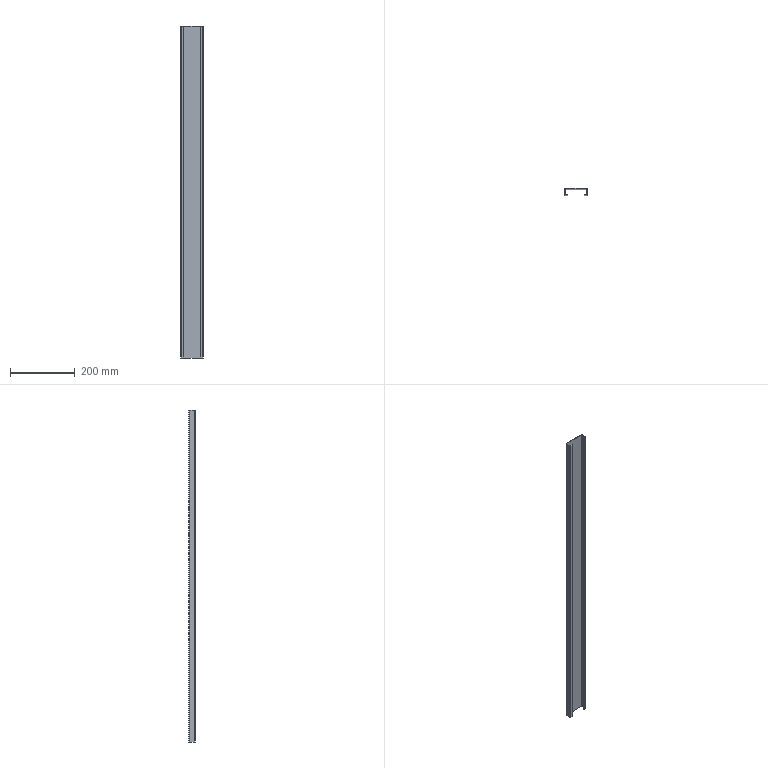Component | SolidWorks | MiddleColumn3-1 | 1 solid | 38 faces | box 70 x 20 x 1025 mm | volume 184711 mm3 | plane 30 | cylinder 8 | commonest cylinder face diameters 3 x4 6 x4
STEP:
#1=COLOUR_RGB('',0.7922,0.8196,0.9333);
#2=FILL_AREA_STYLE_COLOUR('',#1);
#3=FILL_AREA_STYLE('',(#2));
#4=SURFACE_STYLE_FILL_AREA(#3);
#5=SURFACE_SIDE_STYLE('',(#4));
#6=SURFACE_STYLE_USAGE(.BOTH.,#5);
#7=PRESENTATION_STYLE_ASSIGNMENT((#6));
#8=CARTESIAN_POINT('',(-11.614,-13.549,0.9843));
#9=VERTEX_POINT('',#8);
#10=CARTESIAN_POINT('',(-11.614,-13.49,0.9843));
#11=VERTEX_POINT('',#10);
#12=CARTESIAN_POINT('',(-11.614,-13.549,0.9843));
#13=DIRECTION('',(-0.,1.,0.));
#14=VECTOR('',#13,39.37);
#15=LINE('',#12,#14);
#16=EDGE_CURVE('',#9,#11,#15,.T.);
#17=ORIENTED_EDGE('',*,*,#16,.F.);
#18=CARTESIAN_POINT('',(-11.732,-13.431,0.9843));
#19=VERTEX_POINT('',#18);
#20=CARTESIAN_POINT('',(-11.614,-13.431,0.9843));
#21=DIRECTION('',(0.,0.,-1.));
#22=DIRECTION('',(0.,-1.,-0.));
#23=AXIS2_PLACEMENT_3D('',#20,#21,#22);
#24=CIRCLE('',#23,0.1181);
#25=EDGE_CURVE('',#9,#19,#24,.T.);
#26=ORIENTED_EDGE('',*,*,#25,.T.);
#27=CARTESIAN_POINT('',(-11.673,-13.431,0.9843));
#28=VERTEX_POINT('',#27);
#29=CARTESIAN_POINT('',(-11.673,-13.431,0.9843));
#30=DIRECTION('',(-1.,-0.,-0.));
#31=VECTOR('',#30,39.37);
#32=LINE('',#29,#31);
#33=EDGE_CURVE('',#28,#19,#32,.T.);
#34=ORIENTED_EDGE('',*,*,#33,.F.);
#35=CARTESIAN_POINT('',(-11.614,-13.431,0.9843));
#36=DIRECTION('',(0.,0.,-1.));
#37=DIRECTION('',(1.,0.,0.));
#38=AXIS2_PLACEMENT_3D('',#35,#36,#37);
#39=CIRCLE('',#38,0.05906);
#40=EDGE_CURVE('',#11,#28,#39,.T.);
#41=ORIENTED_EDGE('',*,*,#40,.F.);
#42=EDGE_LOOP('',(#17,#26,#34,#41));
#43=FACE_OUTER_BOUND('',#42,.T.);
#44=CARTESIAN_POINT('',(-11.614,-13.549,0.9843));
#45=DIRECTION('',(0.,0.,-1.));
#46=DIRECTION('',(-0.,1.,0.));
#47=AXIS2_PLACEMENT_3D('',#44,#45,#46);
#48=PLANE('',#47);
#49=ADVANCED_FACE('',(#43),#48,.T.);
#50=CARTESIAN_POINT('',(-11.339,-13.549,0.9843));
#51=VERTEX_POINT('',#50);
#52=CARTESIAN_POINT('',(-11.339,-13.549,0.9843));
#53=DIRECTION('',(-1.,-0.,-0.));
#54=VECTOR('',#53,39.37);
#55=LINE('',#52,#54);
#56=EDGE_CURVE('',#51,#9,#55,.T.);
#57=ORIENTED_EDGE('',*,*,#56,.T.);
#58=ORIENTED_EDGE('',*,*,#16,.T.);
#59=CARTESIAN_POINT('',(-11.339,-13.49,0.9843));
#60=VERTEX_POINT('',#59);
#61=CARTESIAN_POINT('',(-11.339,-13.49,0.9843));
#62=DIRECTION('',(-1.,-0.,-0.));
#63=VECTOR('',#62,39.37);
#64=LINE('',#61,#63);
#65=EDGE_CURVE('',#60,#11,#64,.T.);
#66=ORIENTED_EDGE('',*,*,#65,.F.);
#67=CARTESIAN_POINT('',(-11.339,-13.549,0.9843));
#68=DIRECTION('',(-0.,1.,0.));
#69=VECTOR('',#68,39.37);
#70=LINE('',#67,#69);
#71=EDGE_CURVE('',#51,#60,#70,.T.);
#72=ORIENTED_EDGE('',*,*,#71,.F.);
#73=EDGE_LOOP('',(#57,#58,#66,#72));
#74=FACE_OUTER_BOUND('',#73,.T.);
#75=CARTESIAN_POINT('',(-11.673,-13.431,0.9843));
#76=DIRECTION('',(0.,0.,-1.));
#77=DIRECTION('',(-0.,1.,0.));
#78=AXIS2_PLACEMENT_3D('',#75,#76,#77);
#79=PLANE('',#78);
#80=ADVANCED_FACE('',(#74),#79,.T.);
#81=CARTESIAN_POINT('',(-11.732,-13.431,41.339));
#82=VERTEX_POINT('',#81);
#83=CARTESIAN_POINT('',(-11.673,-13.431,41.339));
#84=VERTEX_POINT('',#83);
#85=CARTESIAN_POINT('',(-11.732,-13.431,41.339));
#86=DIRECTION('',(1.,0.,0.));
#87=VECTOR('',#86,39.37);
#88=LINE('',#85,#87);
#89=EDGE_CURVE('',#82,#84,#88,.T.);
#90=ORIENTED_EDGE('',*,*,#89,.F.);
#91=CARTESIAN_POINT('',(-11.614,-13.549,41.339));
#92=VERTEX_POINT('',#91);
#93=CARTESIAN_POINT('',(-11.614,-13.431,41.339));
#94=DIRECTION('',(0.,0.,-1.));
#95=DIRECTION('',(0.,-1.,0.));
#96=AXIS2_PLACEMENT_3D('',#93,#94,#95);
#97=CIRCLE('',#96,0.1181);
#98=EDGE_CURVE('',#92,#82,#97,.T.);
#99=ORIENTED_EDGE('',*,*,#98,.F.);
#100=CARTESIAN_POINT('',(-11.614,-13.49,41.339));
#101=VERTEX_POINT('',#100);
#102=CARTESIAN_POINT('',(-11.614,-13.49,41.339));
#103=DIRECTION('',(0.,-1.,-0.));
#104=VECTOR('',#103,39.37);
#105=LINE('',#102,#104);
#106=EDGE_CURVE('',#101,#92,#105,.T.);
#107=ORIENTED_EDGE('',*,*,#106,.F.);
#108=CARTESIAN_POINT('',(-11.614,-13.431,41.339));
#109=DIRECTION('',(0.,0.,-1.));
#110=DIRECTION('',(1.,0.,0.));
#111=AXIS2_PLACEMENT_3D('',#108,#109,#110);
#112=CIRCLE('',#111,0.05906);
#113=EDGE_CURVE('',#101,#84,#112,.T.);
#114=ORIENTED_EDGE('',*,*,#113,.T.);
#115=EDGE_LOOP('',(#90,#99,#107,#114));
#116=FACE_OUTER_BOUND('',#115,.T.);
#117=CARTESIAN_POINT('',(-11.732,-13.431,41.339));
#118=DIRECTION('',(-0.,-0.,1.));
#119=DIRECTION('',(0.,-1.,-0.));
#120=AXIS2_PLACEMENT_3D('',#117,#118,#119);
#121=PLANE('',#120);
#122=ADVANCED_FACE('',(#116),#121,.T.);
#123=CARTESIAN_POINT('',(-11.732,-12.88,41.339));
#124=VERTEX_POINT('',#123);
#125=CARTESIAN_POINT('',(-11.732,-13.549,41.339));
#126=DIRECTION('',(-0.,1.,0.));
#127=VECTOR('',#126,39.37);
#128=LINE('',#125,#127);
#129=EDGE_CURVE('',#82,#124,#128,.T.);
#130=ORIENTED_EDGE('',*,*,#129,.F.);
#131=ORIENTED_EDGE('',*,*,#89,.T.);
#132=CARTESIAN_POINT('',(-11.673,-12.88,41.339));
#133=VERTEX_POINT('',#132);
#134=CARTESIAN_POINT('',(-11.673,-13.549,41.339));
#135=DIRECTION('',(-0.,1.,0.));
#136=VECTOR('',#135,39.37);
#137=LINE('',#134,#136);
#138=EDGE_CURVE('',#84,#133,#137,.T.);
#139=ORIENTED_EDGE('',*,*,#138,.T.);
#140=CARTESIAN_POINT('',(-11.673,-12.88,41.339));
#141=DIRECTION('',(-1.,0.,-0.));
#142=VECTOR('',#141,39.37);
#143=LINE('',#140,#142);
#144=EDGE_CURVE('',#133,#124,#143,.T.);
#145=ORIENTED_EDGE('',*,*,#144,.T.);
#146=EDGE_LOOP('',(#130,#131,#139,#145));
#147=FACE_OUTER_BOUND('',#146,.T.);
#148=CARTESIAN_POINT('',(-11.614,-13.49,41.339));
#149=DIRECTION('',(-0.,-0.,1.));
#150=DIRECTION('',(0.,-1.,-0.));
#151=AXIS2_PLACEMENT_3D('',#148,#149,#150);
#152=PLANE('',#151);
#153=ADVANCED_FACE('',(#147),#152,.T.);
#154=CARTESIAN_POINT('',(-11.732,-12.88,0.9843));
#155=VERTEX_POINT('',#154);
#156=CARTESIAN_POINT('',(-11.673,-12.88,0.9843));
#157=VERTEX_POINT('',#156);
#158=CARTESIAN_POINT('',(-11.732,-12.88,0.9843));
#159=DIRECTION('',(1.,-0.,0.));
#160=VECTOR('',#159,39.37);
#161=LINE('',#158,#160);
#162=EDGE_CURVE('',#155,#157,#161,.T.);
#163=ORIENTED_EDGE('',*,*,#162,.F.);
#164=CARTESIAN_POINT('',(-11.614,-12.762,0.9843));
#165=VERTEX_POINT('',#164);
#166=CARTESIAN_POINT('',(-11.614,-12.88,0.9843));
#167=DIRECTION('',(0.,0.,-1.));
#168=DIRECTION('',(0.,-1.,-0.));
#169=AXIS2_PLACEMENT_3D('',#166,#167,#168);
#170=CIRCLE('',#169,0.1181);
#171=EDGE_CURVE('',#155,#165,#170,.T.);
#172=ORIENTED_EDGE('',*,*,#171,.T.);
#173=CARTESIAN_POINT('',(-11.614,-12.821,0.9843));
#174=VERTEX_POINT('',#173);
#175=CARTESIAN_POINT('',(-11.614,-12.821,0.9843));
#176=DIRECTION('',(-0.,1.,0.));
#177=VECTOR('',#176,39.37);
#178=LINE('',#175,#177);
#179=EDGE_CURVE('',#174,#165,#178,.T.);
#180=ORIENTED_EDGE('',*,*,#179,.F.);
#181=CARTESIAN_POINT('',(-11.614,-12.88,0.9843));
#182=DIRECTION('',(0.,0.,-1.));
#183=DIRECTION('',(1.,0.,0.));
#184=AXIS2_PLACEMENT_3D('',#181,#182,#183);
#185=CIRCLE('',#184,0.05906);
#186=EDGE_CURVE('',#157,#174,#185,.T.);
#187=ORIENTED_EDGE('',*,*,#186,.F.);
#188=EDGE_LOOP('',(#163,#172,#180,#187));
#189=FACE_OUTER_BOUND('',#188,.T.);
#190=CARTESIAN_POINT('',(-11.732,-12.88,0.9843));
#191=DIRECTION('',(0.,0.,-1.));
#192=DIRECTION('',(-0.,1.,0.));
#193=AXIS2_PLACEMENT_3D('',#190,#191,#192);
#194=PLANE('',#193);
#195=ADVANCED_FACE('',(#189),#194,.T.);
#196=CARTESIAN_POINT('',(-11.732,-13.549,0.9843));
#197=DIRECTION('',(-0.,1.,0.));
#198=VECTOR('',#197,39.37);
#199=LINE('',#196,#198);
#200=EDGE_CURVE('',#19,#155,#199,.T.);
#201=ORIENTED_EDGE('',*,*,#200,.T.);
#202=ORIENTED_EDGE('',*,*,#162,.T.);
#203=CARTESIAN_POINT('',(-11.673,-13.549,0.9843));
#204=DIRECTION('',(-0.,1.,0.));
#205=VECTOR('',#204,39.37);
#206=LINE('',#203,#205);
#207=EDGE_CURVE('',#28,#157,#206,.T.);
#208=ORIENTED_EDGE('',*,*,#207,.F.);
#209=ORIENTED_EDGE('',*,*,#33,.T.);
#210=EDGE_LOOP('',(#201,#202,#208,#209));
#211=FACE_OUTER_BOUND('',#210,.T.);
#212=CARTESIAN_POINT('',(-11.614,-12.821,0.9843));
#213=DIRECTION('',(0.,0.,-1.));
#214=DIRECTION('',(-0.,1.,0.));
#215=AXIS2_PLACEMENT_3D('',#212,#213,#214);
#216=PLANE('',#215);
#217=ADVANCED_FACE('',(#211),#216,.T.);
#218=CARTESIAN_POINT('',(-11.614,-12.762,41.339));
#219=VERTEX_POINT('',#218);
#220=CARTESIAN_POINT('',(-11.614,-12.821,41.339));
#221=VERTEX_POINT('',#220);
#222=CARTESIAN_POINT('',(-11.614,-12.762,41.339));
#223=DIRECTION('',(0.,-1.,-0.));
#224=VECTOR('',#223,39.37);
#225=LINE('',#222,#224);
#226=EDGE_CURVE('',#219,#221,#225,.T.);
#227=ORIENTED_EDGE('',*,*,#226,.F.);
#228=CARTESIAN_POINT('',(-11.614,-12.88,41.339));
#229=DIRECTION('',(0.,0.,-1.));
#230=DIRECTION('',(0.,-1.,0.));
#231=AXIS2_PLACEMENT_3D('',#228,#229,#230);
#232=CIRCLE('',#231,0.1181);
#233=EDGE_CURVE('',#124,#219,#232,.T.);
#234=ORIENTED_EDGE('',*,*,#233,.F.);
#235=ORIENTED_EDGE('',*,*,#144,.F.);
#236=CARTESIAN_POINT('',(-11.614,-12.88,41.339));
#237=DIRECTION('',(0.,0.,-1.));
#238=DIRECTION('',(1.,0.,0.));
#239=AXIS2_PLACEMENT_3D('',#236,#237,#238);
#240=CIRCLE('',#239,0.05906);
#241=EDGE_CURVE('',#133,#221,#240,.T.);
#242=ORIENTED_EDGE('',*,*,#241,.T.);
#243=EDGE_LOOP('',(#227,#234,#235,#242));
#244=FACE_OUTER_BOUND('',#243,.T.);
#245=CARTESIAN_POINT('',(-11.614,-12.762,41.339));
#246=DIRECTION('',(-0.,-0.,1.));
#247=DIRECTION('',(0.,-1.,-0.));
#248=AXIS2_PLACEMENT_3D('',#245,#246,#247);
#249=PLANE('',#248);
#250=ADVANCED_FACE('',(#244),#249,.T.);
#251=CARTESIAN_POINT('',(-9.095,-12.762,41.339));
#252=VERTEX_POINT('',#251);
#253=CARTESIAN_POINT('',(-11.732,-12.762,41.339));
#254=DIRECTION('',(1.,-0.,0.));
#255=VECTOR('',#254,39.37);
#256=LINE('',#253,#255);
#257=EDGE_CURVE('',#219,#252,#256,.T.);
#258=ORIENTED_EDGE('',*,*,#257,.F.);
#259=ORIENTED_EDGE('',*,*,#226,.T.);
#260=CARTESIAN_POINT('',(-9.095,-12.821,41.339));
#261=VERTEX_POINT('',#260);
#262=CARTESIAN_POINT('',(-11.732,-12.821,41.339));
#263=DIRECTION('',(1.,-0.,0.));
#264=VECTOR('',#263,39.37);
#265=LINE('',#262,#264);
#266=EDGE_CURVE('',#221,#261,#265,.T.);
#267=ORIENTED_EDGE('',*,*,#266,.T.);
#268=CARTESIAN_POINT('',(-9.095,-12.821,41.339));
#269=DIRECTION('',(-0.,1.,0.));
#270=VECTOR('',#269,39.37);
#271=LINE('',#268,#270);
#272=EDGE_CURVE('',#261,#252,#271,.T.);
#273=ORIENTED_EDGE('',*,*,#272,.T.);
#274=EDGE_LOOP('',(#258,#259,#267,#273));
#275=FACE_OUTER_BOUND('',#274,.T.);
#276=CARTESIAN_POINT('',(-11.673,-12.88,41.339));
#277=DIRECTION('',(-0.,-0.,1.));
#278=DIRECTION('',(0.,-1.,-0.));
#279=AXIS2_PLACEMENT_3D('',#276,#277,#278);
#280=PLANE('',#279);
#281=ADVANCED_FACE('',(#275),#280,.T.);
#282=CARTESIAN_POINT('',(-9.095,-12.762,0.9843));
#283=VERTEX_POINT('',#282);
#284=CARTESIAN_POINT('',(-9.095,-12.821,0.9843));
#285=VERTEX_POINT('',#284);
#286=CARTESIAN_POINT('',(-9.095,-12.762,0.9843));
#287=DIRECTION('',(0.,-1.,-0.));
#288=VECTOR('',#287,39.37);
#289=LINE('',#286,#288);
#290=EDGE_CURVE('',#283,#285,#289,.T.);
#291=ORIENTED_EDGE('',*,*,#290,.F.);
#292=CARTESIAN_POINT('',(-8.976,-12.88,0.9843));
#293=VERTEX_POINT('',#292);
#294=CARTESIAN_POINT('',(-9.095,-12.88,0.9843));
#295=DIRECTION('',(0.,0.,-1.));
#296=DIRECTION('',(0.,-1.,-0.));
#297=AXIS2_PLACEMENT_3D('',#294,#295,#296);
#298=CIRCLE('',#297,0.1181);
#299=EDGE_CURVE('',#283,#293,#298,.T.);
#300=ORIENTED_EDGE('',*,*,#299,.T.);
#301=CARTESIAN_POINT('',(-9.036,-12.88,0.9843));
#302=VERTEX_POINT('',#301);
#303=CARTESIAN_POINT('',(-9.036,-12.88,0.9843));
#304=DIRECTION('',(1.,0.,0.));
#305=VECTOR('',#304,39.37);
#306=LINE('',#303,#305);
#307=EDGE_CURVE('',#302,#293,#306,.T.);
#308=ORIENTED_EDGE('',*,*,#307,.F.);
#309=CARTESIAN_POINT('',(-9.095,-12.88,0.9843));
#310=DIRECTION('',(0.,0.,-1.));
#311=DIRECTION('',(1.,0.,0.));
#312=AXIS2_PLACEMENT_3D('',#309,#310,#311);
#313=CIRCLE('',#312,0.05906);
#314=EDGE_CURVE('',#285,#302,#313,.T.);
#315=ORIENTED_EDGE('',*,*,#314,.F.);
#316=EDGE_LOOP('',(#291,#300,#308,#315));
#317=FACE_OUTER_BOUND('',#316,.T.);
#318=CARTESIAN_POINT('',(-9.095,-12.762,0.9843));
#319=DIRECTION('',(0.,0.,-1.));
#320=DIRECTION('',(-0.,1.,0.));
#321=AXIS2_PLACEMENT_3D('',#318,#319,#320);
#322=PLANE('',#321);
#323=ADVANCED_FACE('',(#317),#322,.T.);
#324=CARTESIAN_POINT('',(-11.732,-12.762,0.9843));
#325=DIRECTION('',(1.,-0.,0.));
#326=VECTOR('',#325,39.37);
#327=LINE('',#324,#326);
#328=EDGE_CURVE('',#165,#283,#327,.T.);
#329=ORIENTED_EDGE('',*,*,#328,.T.);
#330=ORIENTED_EDGE('',*,*,#290,.T.);
#331=CARTESIAN_POINT('',(-11.732,-12.821,0.9843));
#332=DIRECTION('',(1.,-0.,0.));
#333=VECTOR('',#332,39.37);
#334=LINE('',#331,#333);
#335=EDGE_CURVE('',#174,#285,#334,.T.);
#336=ORIENTED_EDGE('',*,*,#335,.F.);
#337=ORIENTED_EDGE('',*,*,#179,.T.);
#338=EDGE_LOOP('',(#329,#330,#336,#337));
#339=FACE_OUTER_BOUND('',#338,.T.);
#340=CARTESIAN_POINT('',(-9.036,-12.88,0.9843));
#341=DIRECTION('',(0.,0.,-1.));
#342=DIRECTION('',(-0.,1.,0.));
#343=AXIS2_PLACEMENT_3D('',#340,#341,#342);
#344=PLANE('',#343);
#345=ADVANCED_FACE('',(#339),#344,.T.);
#346=CARTESIAN_POINT('',(-8.976,-12.88,41.339));
#347=VERTEX_POINT('',#346);
#348=CARTESIAN_POINT('',(-9.036,-12.88,41.339));
#349=VERTEX_POINT('',#348);
#350=CARTESIAN_POINT('',(-8.976,-12.88,41.339));
#351=DIRECTION('',(-1.,-0.,-0.));
#352=VECTOR('',#351,39.37);
#353=LINE('',#350,#352);
#354=EDGE_CURVE('',#347,#349,#353,.T.);
#355=ORIENTED_EDGE('',*,*,#354,.F.);
#356=CARTESIAN_POINT('',(-9.095,-12.88,41.339));
#357=DIRECTION('',(0.,0.,-1.));
#358=DIRECTION('',(0.,-1.,0.));
#359=AXIS2_PLACEMENT_3D('',#356,#357,#358);
#360=CIRCLE('',#359,0.1181);
#361=EDGE_CURVE('',#252,#347,#360,.T.);
#362=ORIENTED_EDGE('',*,*,#361,.F.);
#363=ORIENTED_EDGE('',*,*,#272,.F.);
#364=CARTESIAN_POINT('',(-9.095,-12.88,41.339));
#365=DIRECTION('',(0.,0.,-1.));
#366=DIRECTION('',(1.,0.,0.));
#367=AXIS2_PLACEMENT_3D('',#364,#365,#366);
#368=CIRCLE('',#367,0.05906);
#369=EDGE_CURVE('',#261,#349,#368,.T.);
#370=ORIENTED_EDGE('',*,*,#369,.T.);
#371=EDGE_LOOP('',(#355,#362,#363,#370));
#372=FACE_OUTER_BOUND('',#371,.T.);
#373=CARTESIAN_POINT('',(-8.976,-12.88,41.339));
#374=DIRECTION('',(-0.,-0.,1.));
#375=DIRECTION('',(0.,-1.,-0.));
#376=AXIS2_PLACEMENT_3D('',#373,#374,#375);
#377=PLANE('',#376);
#378=ADVANCED_FACE('',(#372),#377,.T.);
#379=CARTESIAN_POINT('',(-8.976,-13.431,41.339));
#380=VERTEX_POINT('',#379);
#381=CARTESIAN_POINT('',(-8.976,-12.762,41.339));
#382=DIRECTION('',(0.,-1.,-0.));
#383=VECTOR('',#382,39.37);
#384=LINE('',#381,#383);
#385=EDGE_CURVE('',#347,#380,#384,.T.);
#386=ORIENTED_EDGE('',*,*,#385,.F.);
#387=ORIENTED_EDGE('',*,*,#354,.T.);
#388=CARTESIAN_POINT('',(-9.036,-13.431,41.339));
#389=VERTEX_POINT('',#388);
#390=CARTESIAN_POINT('',(-9.036,-12.762,41.339));
#391=DIRECTION('',(0.,-1.,-0.));
#392=VECTOR('',#391,39.37);
#393=LINE('',#390,#392);
#394=EDGE_CURVE('',#349,#389,#393,.T.);
#395=ORIENTED_EDGE('',*,*,#394,.T.);
#396=CARTESIAN_POINT('',(-9.036,-13.431,41.339));
#397=DIRECTION('',(1.,0.,0.));
#398=VECTOR('',#397,39.37);
#399=LINE('',#396,#398);
#400=EDGE_CURVE('',#389,#380,#399,.T.);
#401=ORIENTED_EDGE('',*,*,#400,.T.);
#402=EDGE_LOOP('',(#386,#387,#395,#401));
#403=FACE_OUTER_BOUND('',#402,.T.);
#404=CARTESIAN_POINT('',(-9.095,-12.821,41.339));
#405=DIRECTION('',(-0.,-0.,1.));
#406=DIRECTION('',(0.,-1.,-0.));
#407=AXIS2_PLACEMENT_3D('',#404,#405,#406);
#408=PLANE('',#407);
#409=ADVANCED_FACE('',(#403),#408,.T.);
#410=CARTESIAN_POINT('',(-8.976,-13.431,0.9843));
#411=VERTEX_POINT('',#410);
#412=CARTESIAN_POINT('',(-9.036,-13.431,0.9843));
#413=VERTEX_POINT('',#412);
#414=CARTESIAN_POINT('',(-8.976,-13.431,0.9843));
#415=DIRECTION('',(-1.,-0.,-0.));
#416=VECTOR('',#415,39.37);
#417=LINE('',#414,#416);
#418=EDGE_CURVE('',#411,#413,#417,.T.);
#419=ORIENTED_EDGE('',*,*,#418,.F.);
#420=CARTESIAN_POINT('',(-9.095,-13.549,0.9843));
#421=VERTEX_POINT('',#420);
#422=CARTESIAN_POINT('',(-9.095,-13.431,0.9843));
#423=DIRECTION('',(0.,0.,-1.));
#424=DIRECTION('',(0.,-1.,-0.));
#425=AXIS2_PLACEMENT_3D('',#422,#423,#424);
#426=CIRCLE('',#425,0.1181);
#427=EDGE_CURVE('',#411,#421,#426,.T.);
#428=ORIENTED_EDGE('',*,*,#427,.T.);
#429=CARTESIAN_POINT('',(-9.095,-13.49,0.9843));
#430=VERTEX_POINT('',#429);
#431=CARTESIAN_POINT('',(-9.095,-13.49,0.9843));
#432=DIRECTION('',(0.,-1.,-0.));
#433=VECTOR('',#432,39.37);
#434=LINE('',#431,#433);
#435=EDGE_CURVE('',#430,#421,#434,.T.);
#436=ORIENTED_EDGE('',*,*,#435,.F.);
#437=CARTESIAN_POINT('',(-9.095,-13.431,0.9843));
#438=DIRECTION('',(0.,0.,-1.));
#439=DIRECTION('',(1.,0.,0.));
#440=AXIS2_PLACEMENT_3D('',#437,#438,#439);
#441=CIRCLE('',#440,0.05906);
#442=EDGE_CURVE('',#413,#430,#441,.T.);
#443=ORIENTED_EDGE('',*,*,#442,.F.);
#444=EDGE_LOOP('',(#419,#428,#436,#443));
#445=FACE_OUTER_BOUND('',#444,.T.);
#446=CARTESIAN_POINT('',(-8.976,-13.431,0.9843));
#447=DIRECTION('',(0.,0.,-1.));
#448=DIRECTION('',(-0.,1.,0.));
#449=AXIS2_PLACEMENT_3D('',#446,#447,#448);
#450=PLANE('',#449);
#451=ADVANCED_FACE('',(#445),#450,.T.);
#452=CARTESIAN_POINT('',(-8.976,-12.762,0.9843));
#453=DIRECTION('',(0.,-1.,-0.));
#454=VECTOR('',#453,39.37);
#455=LINE('',#452,#454);
#456=EDGE_CURVE('',#293,#411,#455,.T.);
#457=ORIENTED_EDGE('',*,*,#456,.T.);
#458=ORIENTED_EDGE('',*,*,#418,.T.);
#459=CARTESIAN_POINT('',(-9.036,-12.762,0.9843));
#460=DIRECTION('',(0.,-1.,-0.));
#461=VECTOR('',#460,39.37);
#462=LINE('',#459,#461);
#463=EDGE_CURVE('',#302,#413,#462,.T.);
#464=ORIENTED_EDGE('',*,*,#463,.F.);
#465=ORIENTED_EDGE('',*,*,#307,.T.);
#466=EDGE_LOOP('',(#457,#458,#464,#465));
#467=FACE_OUTER_BOUND('',#466,.T.);
#468=CARTESIAN_POINT('',(-9.095,-13.49,0.9843));
#469=DIRECTION('',(0.,0.,-1.));
#470=DIRECTION('',(-0.,1.,0.));
#471=AXIS2_PLACEMENT_3D('',#468,#469,#470);
#472=PLANE('',#471);
#473=ADVANCED_FACE('',(#467),#472,.T.);
#474=CARTESIAN_POINT('',(-9.095,-13.549,41.339));
#475=VERTEX_POINT('',#474);
#476=CARTESIAN_POINT('',(-9.095,-13.49,41.339));
#477=VERTEX_POINT('',#476);
#478=CARTESIAN_POINT('',(-9.095,-13.549,41.339));
#479=DIRECTION('',(-0.,1.,0.));
#480=VECTOR('',#479,39.37);
#481=LINE('',#478,#480);
#482=EDGE_CURVE('',#475,#477,#481,.T.);
#483=ORIENTED_EDGE('',*,*,#482,.F.);
#484=CARTESIAN_POINT('',(-9.095,-13.431,41.339));
#485=DIRECTION('',(0.,0.,-1.));
#486=DIRECTION('',(0.,-1.,0.));
#487=AXIS2_PLACEMENT_3D('',#484,#485,#486);
#488=CIRCLE('',#487,0.1181);
#489=EDGE_CURVE('',#380,#475,#488,.T.);
#490=ORIENTED_EDGE('',*,*,#489,.F.);
#491=ORIENTED_EDGE('',*,*,#400,.F.);
#492=CARTESIAN_POINT('',(-9.095,-13.431,41.339));
#493=DIRECTION('',(0.,0.,-1.));
#494=DIRECTION('',(1.,0.,0.));
#495=AXIS2_PLACEMENT_3D('',#492,#493,#494);
#496=CIRCLE('',#495,0.05906);
#497=EDGE_CURVE('',#389,#477,#496,.T.);
#498=ORIENTED_EDGE('',*,*,#497,.T.);
#499=EDGE_LOOP('',(#483,#490,#491,#498));
#500=FACE_OUTER_BOUND('',#499,.T.);
#501=CARTESIAN_POINT('',(-9.095,-13.549,41.339));
#502=DIRECTION('',(-0.,-0.,1.));
#503=DIRECTION('',(0.,-1.,-0.));
#504=AXIS2_PLACEMENT_3D('',#501,#502,#503);
#505=PLANE('',#504);
#506=ADVANCED_FACE('',(#500),#505,.T.);
#507=CARTESIAN_POINT('',(-9.37,-13.549,41.339));
#508=VERTEX_POINT('',#507);
#509=CARTESIAN_POINT('',(-8.976,-13.549,41.339));
#510=DIRECTION('',(-1.,-0.,-0.));
#511=VECTOR('',#510,39.37);
#512=LINE('',#509,#511);
#513=EDGE_CURVE('',#475,#508,#512,.T.);
#514=ORIENTED_EDGE('',*,*,#513,.F.);
#515=ORIENTED_EDGE('',*,*,#482,.T.);
#516=CARTESIAN_POINT('',(-9.37,-13.49,41.339));
#517=VERTEX_POINT('',#516);
#518=CARTESIAN_POINT('',(-8.976,-13.49,41.339));
#519=DIRECTION('',(-1.,-0.,-0.));
#520=VECTOR('',#519,39.37);
#521=LINE('',#518,#520);
#522=EDGE_CURVE('',#477,#517,#521,.T.);
#523=ORIENTED_EDGE('',*,*,#522,.T.);
#524=CARTESIAN_POINT('',(-9.37,-13.49,41.339));
#525=DIRECTION('',(0.,-1.,-0.));
#526=VECTOR('',#525,39.37);
#527=LINE('',#524,#526);
#528=EDGE_CURVE('',#517,#508,#527,.T.);
#529=ORIENTED_EDGE('',*,*,#528,.T.);
#530=EDGE_LOOP('',(#514,#515,#523,#529));
#531=FACE_OUTER_BOUND('',#530,.T.);
#532=CARTESIAN_POINT('',(-9.036,-13.431,41.339));
#533=DIRECTION('',(-0.,-0.,1.));
#534=DIRECTION('',(0.,-1.,-0.));
#535=AXIS2_PLACEMENT_3D('',#532,#533,#534);
#536=PLANE('',#535);
#537=ADVANCED_FACE('',(#531),#536,.T.);
#538=ORIENTED_EDGE('',*,*,#513,.T.);
#539=CARTESIAN_POINT('',(-9.37,-13.549,0.9843));
#540=VERTEX_POINT('',#539);
#541=CARTESIAN_POINT('',(-9.37,-13.549,0.9843));
#542=DIRECTION('',(-0.,-0.,1.));
#543=VECTOR('',#542,39.37);
#544=LINE('',#541,#543);
#545=EDGE_CURVE('',#540,#508,#544,.T.);
#546=ORIENTED_EDGE('',*,*,#545,.F.);
#547=CARTESIAN_POINT('',(-8.976,-13.549,0.9843));
#548=DIRECTION('',(-1.,-0.,-0.));
#549=VECTOR('',#548,39.37);
#550=LINE('',#547,#549);
#551=EDGE_CURVE('',#421,#540,#550,.T.);
#552=ORIENTED_EDGE('',*,*,#551,.F.);
#553=CARTESIAN_POINT('',(-9.095,-13.549,0.9843));
#554=DIRECTION('',(-0.,-0.,1.));
#555=VECTOR('',#554,39.37);
#556=LINE('',#553,#555);
#557=EDGE_CURVE('',#421,#475,#556,.T.);
#558=ORIENTED_EDGE('',*,*,#557,.T.);
#559=EDGE_LOOP('',(#538,#546,#552,#558));
#560=FACE_OUTER_BOUND('',#559,.T.);
#561=CARTESIAN_POINT('',(-8.976,-13.549,0.9843));
#562=DIRECTION('',(-0.,1.,0.));
#563=DIRECTION('',(1.,0.,0.));
#564=AXIS2_PLACEMENT_3D('',#561,#562,#563);
#565=PLANE('',#564);
#566=ADVANCED_FACE('',(#560),#565,.F.);
#567=ORIENTED_EDGE('',*,*,#528,.F.);
#568=CARTESIAN_POINT('',(-9.37,-13.49,0.9843));
#569=VERTEX_POINT('',#568);
#570=CARTESIAN_POINT('',(-9.37,-13.49,0.9843));
#571=DIRECTION('',(-0.,-0.,1.));
#572=VECTOR('',#571,39.37);
#573=LINE('',#570,#572);
#574=EDGE_CURVE('',#569,#517,#573,.T.);
#575=ORIENTED_EDGE('',*,*,#574,.F.);
#576=CARTESIAN_POINT('',(-9.37,-13.49,0.9843));
#577=DIRECTION('',(0.,-1.,-0.));
#578=VECTOR('',#577,39.37);
#579=LINE('',#576,#578);
#580=EDGE_CURVE('',#569,#540,#579,.T.);
#581=ORIENTED_EDGE('',*,*,#580,.T.);
#582=ORIENTED_EDGE('',*,*,#545,.T.);
#583=EDGE_LOOP('',(#567,#575,#581,#582));
#584=FACE_OUTER_BOUND('',#583,.T.);
#585=CARTESIAN_POINT('',(-9.37,-13.49,0.9843));
#586=DIRECTION('',(-1.,-0.,-0.));
#587=DIRECTION('',(-0.,1.,0.));
#588=AXIS2_PLACEMENT_3D('',#585,#586,#587);
#589=PLANE('',#588);
#590=ADVANCED_FACE('',(#584),#589,.T.);
#591=ORIENTED_EDGE('',*,*,#522,.F.);
#592=CARTESIAN_POINT('',(-9.095,-13.49,0.9843));
#593=DIRECTION('',(-0.,-0.,1.));
#594=VECTOR('',#593,39.37);
#595=LINE('',#592,#594);
#596=EDGE_CURVE('',#430,#477,#595,.T.);
#597=ORIENTED_EDGE('',*,*,#596,.F.);
#598=CARTESIAN_POINT('',(-8.976,-13.49,0.9843));
#599=DIRECTION('',(-1.,-0.,-0.));
#600=VECTOR('',#599,39.37);
#601=LINE('',#598,#600);
#602=EDGE_CURVE('',#430,#569,#601,.T.);
#603=ORIENTED_EDGE('',*,*,#602,.T.);
#604=ORIENTED_EDGE('',*,*,#574,.T.);
#605=EDGE_LOOP('',(#591,#597,#603,#604));
#606=FACE_OUTER_BOUND('',#605,.T.);
#607=CARTESIAN_POINT('',(-8.976,-13.49,0.9843));
#608=DIRECTION('',(-0.,1.,0.));
#609=DIRECTION('',(1.,0.,0.));
#610=AXIS2_PLACEMENT_3D('',#607,#608,#609);
#611=PLANE('',#610);
#612=ADVANCED_FACE('',(#606),#611,.T.);
#613=ORIENTED_EDGE('',*,*,#497,.F.);
#614=CARTESIAN_POINT('',(-9.036,-13.431,0.9843));
#615=DIRECTION('',(-0.,-0.,1.));
#616=VECTOR('',#615,39.37);
#617=LINE('',#614,#616);
#618=EDGE_CURVE('',#413,#389,#617,.T.);
#619=ORIENTED_EDGE('',*,*,#618,.F.);
#620=ORIENTED_EDGE('',*,*,#442,.T.);
#621=ORIENTED_EDGE('',*,*,#596,.T.);
#622=EDGE_LOOP('',(#613,#619,#620,#621));
#623=FACE_OUTER_BOUND('',#622,.T.);
#624=CARTESIAN_POINT('',(-9.095,-13.431,0.9843));
#625=DIRECTION('',(-0.,-0.,1.));
#626=DIRECTION('',(0.,-1.,-0.));
#627=AXIS2_PLACEMENT_3D('',#624,#625,#626);
#628=CYLINDRICAL_SURFACE('',#627,0.05906);
#629=ADVANCED_FACE('',(#623),#628,.F.);
#630=ORIENTED_EDGE('',*,*,#394,.F.);
#631=CARTESIAN_POINT('',(-9.036,-12.88,0.9843));
#632=DIRECTION('',(-0.,-0.,1.));
#633=VECTOR('',#632,39.37);
#634=LINE('',#631,#633);
#635=EDGE_CURVE('',#302,#349,#634,.T.);
#636=ORIENTED_EDGE('',*,*,#635,.F.);
#637=ORIENTED_EDGE('',*,*,#463,.T.);
#638=ORIENTED_EDGE('',*,*,#618,.T.);
#639=EDGE_LOOP('',(#630,#636,#637,#638));
#640=FACE_OUTER_BOUND('',#639,.T.);
#641=CARTESIAN_POINT('',(-9.036,-12.762,0.9843));
#642=DIRECTION('',(-1.,-0.,-0.));
#643=DIRECTION('',(-0.,1.,0.));
#644=AXIS2_PLACEMENT_3D('',#641,#642,#643);
#645=PLANE('',#644);
#646=ADVANCED_FACE('',(#640),#645,.T.);
#647=ORIENTED_EDGE('',*,*,#369,.F.);
#648=CARTESIAN_POINT('',(-9.095,-12.821,0.9843));
#649=DIRECTION('',(-0.,-0.,1.));
#650=VECTOR('',#649,39.37);
#651=LINE('',#648,#650);
#652=EDGE_CURVE('',#285,#261,#651,.T.);
#653=ORIENTED_EDGE('',*,*,#652,.F.);
#654=ORIENTED_EDGE('',*,*,#314,.T.);
#655=ORIENTED_EDGE('',*,*,#635,.T.);
#656=EDGE_LOOP('',(#647,#653,#654,#655));
#657=FACE_OUTER_BOUND('',#656,.T.);
#658=CARTESIAN_POINT('',(-9.095,-12.88,0.9843));
#659=DIRECTION('',(-0.,-0.,1.));
#660=DIRECTION('',(0.,-1.,-0.));
#661=AXIS2_PLACEMENT_3D('',#658,#659,#660);
#662=CYLINDRICAL_SURFACE('',#661,0.05906);
#663=ADVANCED_FACE('',(#657),#662,.F.);
#664=ORIENTED_EDGE('',*,*,#266,.F.);
#665=CARTESIAN_POINT('',(-11.614,-12.821,0.9843));
#666=DIRECTION('',(-0.,-0.,1.));
#667=VECTOR('',#666,39.37);
#668=LINE('',#665,#667);
#669=EDGE_CURVE('',#174,#221,#668,.T.);
#670=ORIENTED_EDGE('',*,*,#669,.F.);
#671=ORIENTED_EDGE('',*,*,#335,.T.);
#672=ORIENTED_EDGE('',*,*,#652,.T.);
#673=EDGE_LOOP('',(#664,#670,#671,#672));
#674=FACE_OUTER_BOUND('',#673,.T.);
#675=CARTESIAN_POINT('',(-11.732,-12.821,0.9843));
#676=DIRECTION('',(-0.,-1.,-0.));
#677=DIRECTION('',(-1.,0.,-0.));
#678=AXIS2_PLACEMENT_3D('',#675,#676,#677);
#679=PLANE('',#678);
#680=ADVANCED_FACE('',(#674),#679,.T.);
#681=ORIENTED_EDGE('',*,*,#241,.F.);
#682=CARTESIAN_POINT('',(-11.673,-12.88,0.9843));
#683=DIRECTION('',(-0.,-0.,1.));
#684=VECTOR('',#683,39.37);
#685=LINE('',#682,#684);
#686=EDGE_CURVE('',#157,#133,#685,.T.);
#687=ORIENTED_EDGE('',*,*,#686,.F.);
#688=ORIENTED_EDGE('',*,*,#186,.T.);
#689=ORIENTED_EDGE('',*,*,#669,.T.);
#690=EDGE_LOOP('',(#681,#687,#688,#689));
#691=FACE_OUTER_BOUND('',#690,.T.);
#692=CARTESIAN_POINT('',(-11.614,-12.88,0.9843));
#693=DIRECTION('',(-0.,-0.,1.));
#694=DIRECTION('',(0.,-1.,-0.));
#695=AXIS2_PLACEMENT_3D('',#692,#693,#694);
#696=CYLINDRICAL_SURFACE('',#695,0.05906);
#697=ADVANCED_FACE('',(#691),#696,.F.);
#698=ORIENTED_EDGE('',*,*,#138,.F.);
#699=CARTESIAN_POINT('',(-11.673,-13.431,0.9843));
#700=DIRECTION('',(-0.,-0.,1.));
#701=VECTOR('',#700,39.37);
#702=LINE('',#699,#701);
#703=EDGE_CURVE('',#28,#84,#702,.T.);
#704=ORIENTED_EDGE('',*,*,#703,.F.);
#705=ORIENTED_EDGE('',*,*,#207,.T.);
#706=ORIENTED_EDGE('',*,*,#686,.T.);
#707=EDGE_LOOP('',(#698,#704,#705,#706));
#708=FACE_OUTER_BOUND('',#707,.T.);
#709=CARTESIAN_POINT('',(-11.673,-13.549,0.9843));
#710=DIRECTION('',(1.,0.,0.));
#711=DIRECTION('',(0.,-1.,-0.));
#712=AXIS2_PLACEMENT_3D('',#709,#710,#711);
#713=PLANE('',#712);
#714=ADVANCED_FACE('',(#708),#713,.T.);
#715=ORIENTED_EDGE('',*,*,#113,.F.);
#716=CARTESIAN_POINT('',(-11.614,-13.49,0.9843));
#717=DIRECTION('',(-0.,-0.,1.));
#718=VECTOR('',#717,39.37);
#719=LINE('',#716,#718);
#720=EDGE_CURVE('',#11,#101,#719,.T.);
#721=ORIENTED_EDGE('',*,*,#720,.F.);
#722=ORIENTED_EDGE('',*,*,#40,.T.);
#723=ORIENTED_EDGE('',*,*,#703,.T.);
#724=EDGE_LOOP('',(#715,#721,#722,#723));
#725=FACE_OUTER_BOUND('',#724,.T.);
#726=CARTESIAN_POINT('',(-11.614,-13.431,0.9843));
#727=DIRECTION('',(-0.,-0.,1.));
#728=DIRECTION('',(0.,-1.,-0.));
#729=AXIS2_PLACEMENT_3D('',#726,#727,#728);
#730=CYLINDRICAL_SURFACE('',#729,0.05906);
#731=ADVANCED_FACE('',(#725),#730,.F.);
#732=CARTESIAN_POINT('',(-11.339,-13.49,41.339));
#733=VERTEX_POINT('',#732);
#734=CARTESIAN_POINT('',(-11.339,-13.49,41.339));
#735=DIRECTION('',(-1.,-0.,-0.));
#736=VECTOR('',#735,39.37);
#737=LINE('',#734,#736);
#738=EDGE_CURVE('',#733,#101,#737,.T.);
#739=ORIENTED_EDGE('',*,*,#738,.F.);
#740=CARTESIAN_POINT('',(-11.339,-13.49,0.9843));
#741=DIRECTION('',(-0.,-0.,1.));
#742=VECTOR('',#741,39.37);
#743=LINE('',#740,#742);
#744=EDGE_CURVE('',#60,#733,#743,.T.);
#745=ORIENTED_EDGE('',*,*,#744,.F.);
#746=ORIENTED_EDGE('',*,*,#65,.T.);
#747=ORIENTED_EDGE('',*,*,#720,.T.);
#748=EDGE_LOOP('',(#739,#745,#746,#747));
#749=FACE_OUTER_BOUND('',#748,.T.);
#750=CARTESIAN_POINT('',(-11.339,-13.49,0.9843));
#751=DIRECTION('',(-0.,1.,0.));
#752=DIRECTION('',(1.,0.,0.));
#753=AXIS2_PLACEMENT_3D('',#750,#751,#752);
#754=PLANE('',#753);
#755=ADVANCED_FACE('',(#749),#754,.T.);
#756=CARTESIAN_POINT('',(-11.339,-13.549,41.339));
#757=VERTEX_POINT('',#756);
#758=CARTESIAN_POINT('',(-11.339,-13.549,41.339));
#759=DIRECTION('',(-0.,1.,0.));
#760=VECTOR('',#759,39.37);
#761=LINE('',#758,#760);
#762=EDGE_CURVE('',#757,#733,#761,.T.);
#763=ORIENTED_EDGE('',*,*,#762,.F.);
#764=CARTESIAN_POINT('',(-11.339,-13.549,0.9843));
#765=DIRECTION('',(-0.,-0.,1.));
#766=VECTOR('',#765,39.37);
#767=LINE('',#764,#766);
#768=EDGE_CURVE('',#51,#757,#767,.T.);
#769=ORIENTED_EDGE('',*,*,#768,.F.);
#770=ORIENTED_EDGE('',*,*,#71,.T.);
#771=ORIENTED_EDGE('',*,*,#744,.T.);
#772=EDGE_LOOP('',(#763,#769,#770,#771));
#773=FACE_OUTER_BOUND('',#772,.T.);
#774=CARTESIAN_POINT('',(-11.339,-13.549,0.9843));
#775=DIRECTION('',(1.,0.,0.));
#776=DIRECTION('',(0.,-1.,-0.));
#777=AXIS2_PLACEMENT_3D('',#774,#775,#776);
#778=PLANE('',#777);
#779=ADVANCED_FACE('',(#773),#778,.T.);
#780=CARTESIAN_POINT('',(-11.339,-13.549,41.339));
#781=DIRECTION('',(-1.,-0.,-0.));
#782=VECTOR('',#781,39.37);
#783=LINE('',#780,#782);
#784=EDGE_CURVE('',#757,#92,#783,.T.);
#785=ORIENTED_EDGE('',*,*,#784,.T.);
#786=CARTESIAN_POINT('',(-11.614,-13.549,0.9843));
#787=DIRECTION('',(-0.,-0.,1.));
#788=VECTOR('',#787,39.37);
#789=LINE('',#786,#788);
#790=EDGE_CURVE('',#9,#92,#789,.T.);
#791=ORIENTED_EDGE('',*,*,#790,.F.);
#792=ORIENTED_EDGE('',*,*,#56,.F.);
#793=ORIENTED_EDGE('',*,*,#768,.T.);
#794=EDGE_LOOP('',(#785,#791,#792,#793));
#795=FACE_OUTER_BOUND('',#794,.T.);
#796=CARTESIAN_POINT('',(-11.339,-13.549,0.9843));
#797=DIRECTION('',(-0.,1.,0.));
#798=DIRECTION('',(1.,0.,0.));
#799=AXIS2_PLACEMENT_3D('',#796,#797,#798);
#800=PLANE('',#799);
#801=ADVANCED_FACE('',(#795),#800,.F.);
#802=ORIENTED_EDGE('',*,*,#98,.T.);
#803=CARTESIAN_POINT('',(-11.732,-13.431,0.9843));
#804=DIRECTION('',(-0.,-0.,1.));
#805=VECTOR('',#804,39.37);
#806=LINE('',#803,#805);
#807=EDGE_CURVE('',#19,#82,#806,.T.);
#808=ORIENTED_EDGE('',*,*,#807,.F.);
#809=ORIENTED_EDGE('',*,*,#25,.F.);
#810=ORIENTED_EDGE('',*,*,#790,.T.);
#811=EDGE_LOOP('',(#802,#808,#809,#810));
#812=FACE_OUTER_BOUND('',#811,.T.);
#813=CARTESIAN_POINT('',(-11.614,-13.431,0.9843));
#814=DIRECTION('',(-0.,-0.,1.));
#815=DIRECTION('',(0.,-1.,-0.));
#816=AXIS2_PLACEMENT_3D('',#813,#814,#815);
#817=CYLINDRICAL_SURFACE('',#816,0.1181);
#818=ADVANCED_FACE('',(#812),#817,.T.);
#819=ORIENTED_EDGE('',*,*,#129,.T.);
#820=CARTESIAN_POINT('',(-11.732,-12.88,0.9843));
#821=DIRECTION('',(-0.,-0.,1.));
#822=VECTOR('',#821,39.37);
#823=LINE('',#820,#822);
#824=EDGE_CURVE('',#155,#124,#823,.T.);
#825=ORIENTED_EDGE('',*,*,#824,.F.);
#826=ORIENTED_EDGE('',*,*,#200,.F.);
#827=ORIENTED_EDGE('',*,*,#807,.T.);
#828=EDGE_LOOP('',(#819,#825,#826,#827));
#829=FACE_OUTER_BOUND('',#828,.T.);
#830=CARTESIAN_POINT('',(-11.732,-13.549,0.9843));
#831=DIRECTION('',(1.,0.,0.));
#832=DIRECTION('',(0.,-1.,-0.));
#833=AXIS2_PLACEMENT_3D('',#830,#831,#832);
#834=PLANE('',#833);
#835=ADVANCED_FACE('',(#829),#834,.F.);
#836=ORIENTED_EDGE('',*,*,#233,.T.);
#837=CARTESIAN_POINT('',(-11.614,-12.762,0.9843));
#838=DIRECTION('',(-0.,-0.,1.));
#839=VECTOR('',#838,39.37);
#840=LINE('',#837,#839);
#841=EDGE_CURVE('',#165,#219,#840,.T.);
#842=ORIENTED_EDGE('',*,*,#841,.F.);
#843=ORIENTED_EDGE('',*,*,#171,.F.);
#844=ORIENTED_EDGE('',*,*,#824,.T.);
#845=EDGE_LOOP('',(#836,#842,#843,#844));
#846=FACE_OUTER_BOUND('',#845,.T.);
#847=CARTESIAN_POINT('',(-11.614,-12.88,0.9843));
#848=DIRECTION('',(-0.,-0.,1.));
#849=DIRECTION('',(0.,-1.,-0.));
#850=AXIS2_PLACEMENT_3D('',#847,#848,#849);
#851=CYLINDRICAL_SURFACE('',#850,0.1181);
#852=ADVANCED_FACE('',(#846),#851,.T.);
#853=ORIENTED_EDGE('',*,*,#257,.T.);
#854=CARTESIAN_POINT('',(-9.095,-12.762,0.9843));
#855=DIRECTION('',(-0.,-0.,1.));
#856=VECTOR('',#855,39.37);
#857=LINE('',#854,#856);
#858=EDGE_CURVE('',#283,#252,#857,.T.);
#859=ORIENTED_EDGE('',*,*,#858,.F.);
#860=ORIENTED_EDGE('',*,*,#328,.F.);
#861=ORIENTED_EDGE('',*,*,#841,.T.);
#862=EDGE_LOOP('',(#853,#859,#860,#861));
#863=FACE_OUTER_BOUND('',#862,.T.);
#864=CARTESIAN_POINT('',(-11.732,-12.762,0.9843));
#865=DIRECTION('',(-0.,-1.,-0.));
#866=DIRECTION('',(-1.,0.,-0.));
#867=AXIS2_PLACEMENT_3D('',#864,#865,#866);
#868=PLANE('',#867);
#869=ADVANCED_FACE('',(#863),#868,.F.);
#870=ORIENTED_EDGE('',*,*,#361,.T.);
#871=CARTESIAN_POINT('',(-8.976,-12.88,0.9843));
#872=DIRECTION('',(-0.,-0.,1.));
#873=VECTOR('',#872,39.37);
#874=LINE('',#871,#873);
#875=EDGE_CURVE('',#293,#347,#874,.T.);
#876=ORIENTED_EDGE('',*,*,#875,.F.);
#877=ORIENTED_EDGE('',*,*,#299,.F.);
#878=ORIENTED_EDGE('',*,*,#858,.T.);
#879=EDGE_LOOP('',(#870,#876,#877,#878));
#880=FACE_OUTER_BOUND('',#879,.T.);
#881=CARTESIAN_POINT('',(-9.095,-12.88,0.9843));
#882=DIRECTION('',(-0.,-0.,1.));
#883=DIRECTION('',(0.,-1.,-0.));
#884=AXIS2_PLACEMENT_3D('',#881,#882,#883);
#885=CYLINDRICAL_SURFACE('',#884,0.1181);
#886=ADVANCED_FACE('',(#880),#885,.T.);
#887=ORIENTED_EDGE('',*,*,#385,.T.);
#888=CARTESIAN_POINT('',(-8.976,-13.431,0.9843));
#889=DIRECTION('',(-0.,-0.,1.));
#890=VECTOR('',#889,39.37);
#891=LINE('',#888,#890);
#892=EDGE_CURVE('',#411,#380,#891,.T.);
#893=ORIENTED_EDGE('',*,*,#892,.F.);
#894=ORIENTED_EDGE('',*,*,#456,.F.);
#895=ORIENTED_EDGE('',*,*,#875,.T.);
#896=EDGE_LOOP('',(#887,#893,#894,#895));
#897=FACE_OUTER_BOUND('',#896,.T.);
#898=CARTESIAN_POINT('',(-8.976,-12.762,0.9843));
#899=DIRECTION('',(-1.,-0.,-0.));
#900=DIRECTION('',(-0.,1.,0.));
#901=AXIS2_PLACEMENT_3D('',#898,#899,#900);
#902=PLANE('',#901);
#903=ADVANCED_FACE('',(#897),#902,.F.);
#904=ORIENTED_EDGE('',*,*,#489,.T.);
#905=ORIENTED_EDGE('',*,*,#557,.F.);
#906=ORIENTED_EDGE('',*,*,#427,.F.);
#907=ORIENTED_EDGE('',*,*,#892,.T.);
#908=EDGE_LOOP('',(#904,#905,#906,#907));
#909=FACE_OUTER_BOUND('',#908,.T.);
#910=CARTESIAN_POINT('',(-9.095,-13.431,0.9843));
#911=DIRECTION('',(-0.,-0.,1.));
#912=DIRECTION('',(0.,-1.,-0.));
#913=AXIS2_PLACEMENT_3D('',#910,#911,#912);
#914=CYLINDRICAL_SURFACE('',#913,0.1181);
#915=ADVANCED_FACE('',(#909),#914,.T.);
#916=ORIENTED_EDGE('',*,*,#551,.T.);
#917=ORIENTED_EDGE('',*,*,#580,.F.);
#918=ORIENTED_EDGE('',*,*,#602,.F.);
#919=ORIENTED_EDGE('',*,*,#435,.T.);
#920=EDGE_LOOP('',(#916,#917,#918,#919));
#921=FACE_OUTER_BOUND('',#920,.T.);
#922=CARTESIAN_POINT('',(-9.095,-13.431,0.9843));
#923=DIRECTION('',(0.,0.,-1.));
#924=DIRECTION('',(1.,0.,0.));
#925=AXIS2_PLACEMENT_3D('',#922,#923,#924);
#926=PLANE('',#925);
#927=ADVANCED_FACE('',(#921),#926,.T.);
#928=ORIENTED_EDGE('',*,*,#738,.T.);
#929=ORIENTED_EDGE('',*,*,#106,.T.);
#930=ORIENTED_EDGE('',*,*,#784,.F.);
#931=ORIENTED_EDGE('',*,*,#762,.T.);
#932=EDGE_LOOP('',(#928,#929,#930,#931));
#933=FACE_OUTER_BOUND('',#932,.T.);
#934=CARTESIAN_POINT('',(-9.095,-13.431,41.339));
#935=DIRECTION('',(0.,0.,-1.));
#936=DIRECTION('',(1.,0.,0.));
#937=AXIS2_PLACEMENT_3D('',#934,#935,#936);
#938=PLANE('',#937);
#939=ADVANCED_FACE('',(#933),#938,.F.);
#940=CLOSED_SHELL('',(#49,#80,#122,#153,#195,#217,#250,#281,#323,#345,#378,#409,#451,#473,#506,#537,#566,#590,#612,#629,#646,#663,#680,#697,#714,#731,#755,#779,#801,#818,#835,#852,#869,#886,#903,#915,#927,#939));
#941=MANIFOLD_SOLID_BREP('',#940);
#942=STYLED_ITEM('',(#7),#941);
#943=PRESENTATION_LAYER_ASSIGNMENT('','',(#942));
#944=CARTESIAN_POINT('',(0.,0.,0.));
#945=DIRECTION('',(0.,0.,1.));
#946=DIRECTION('',(1.,0.,0.));
#947=AXIS2_PLACEMENT_3D('',#944,#945,#946);
#948=(LENGTH_UNIT()NAMED_UNIT(*)SI_UNIT($,.METRE.));
#949=LENGTH_MEASURE_WITH_UNIT(LENGTH_MEASURE(0.0254),#948);
#950=DIMENSIONAL_EXPONENTS(1.,0.,0.,0.,0.,0.,0.);
#951=(CONVERSION_BASED_UNIT('',#949)LENGTH_UNIT()NAMED_UNIT(#950));
#952=UNCERTAINTY_MEASURE_WITH_UNIT(LENGTH_MEASURE(0.00001),#951,'','');
#953=(NAMED_UNIT(*)PLANE_ANGLE_UNIT()SI_UNIT($,.RADIAN.));
#954=(NAMED_UNIT(*)SI_UNIT($,.STERADIAN.)SOLID_ANGLE_UNIT());
#955=(GEOMETRIC_REPRESENTATION_CONTEXT(3)GLOBAL_UNCERTAINTY_ASSIGNED_CONTEXT((#952))GLOBAL_UNIT_ASSIGNED_CONTEXT((#951,#953,#954))REPRESENTATION_CONTEXT('',''));
#956=ADVANCED_BREP_SHAPE_REPRESENTATION('',(#941,#947),#955);
#957=(LENGTH_UNIT()NAMED_UNIT(*)SI_UNIT($,.METRE.));
#958=LENGTH_MEASURE_WITH_UNIT(LENGTH_MEASURE(0.0254),#957);
#959=DIMENSIONAL_EXPONENTS(1.,0.,0.,0.,0.,0.,0.);
#960=(CONVERSION_BASED_UNIT('',#958)LENGTH_UNIT()NAMED_UNIT(#959));
#961=UNCERTAINTY_MEASURE_WITH_UNIT(LENGTH_MEASURE(0.00001),#960,'','');
#962=(NAMED_UNIT(*)PLANE_ANGLE_UNIT()SI_UNIT($,.RADIAN.));
#963=(NAMED_UNIT(*)SI_UNIT($,.STERADIAN.)SOLID_ANGLE_UNIT());
#964=(GEOMETRIC_REPRESENTATION_CONTEXT(3)GLOBAL_UNCERTAINTY_ASSIGNED_CONTEXT((#961))GLOBAL_UNIT_ASSIGNED_CONTEXT((#960,#962,#963))REPRESENTATION_CONTEXT('',''));
#965=MECHANICAL_DESIGN_GEOMETRIC_PRESENTATION_REPRESENTATION('',(#942),#964);